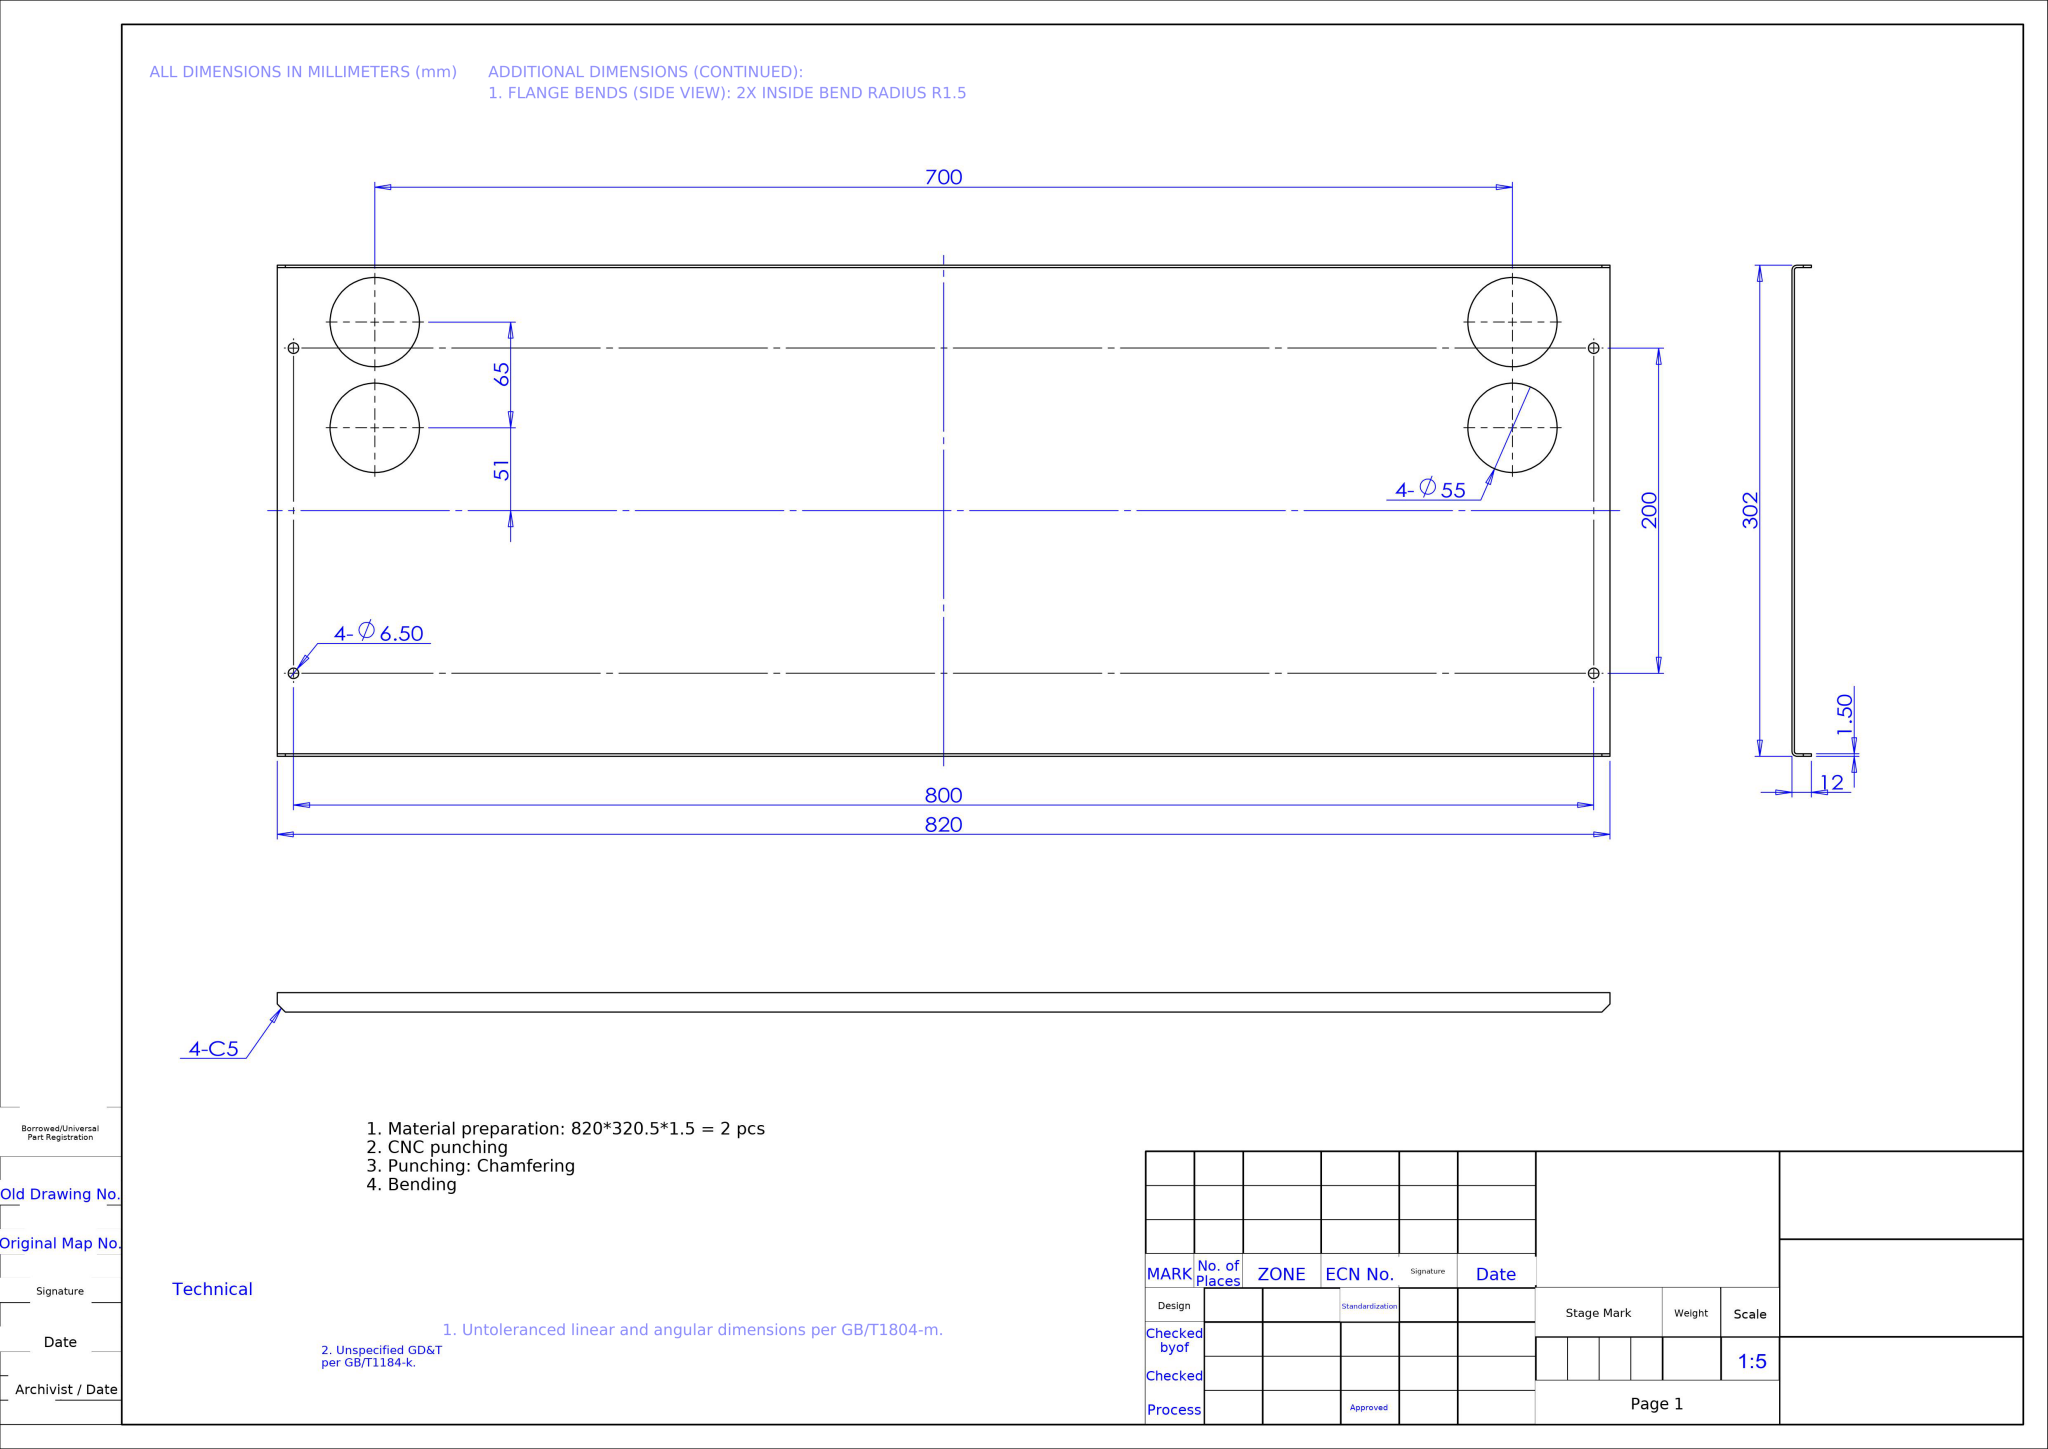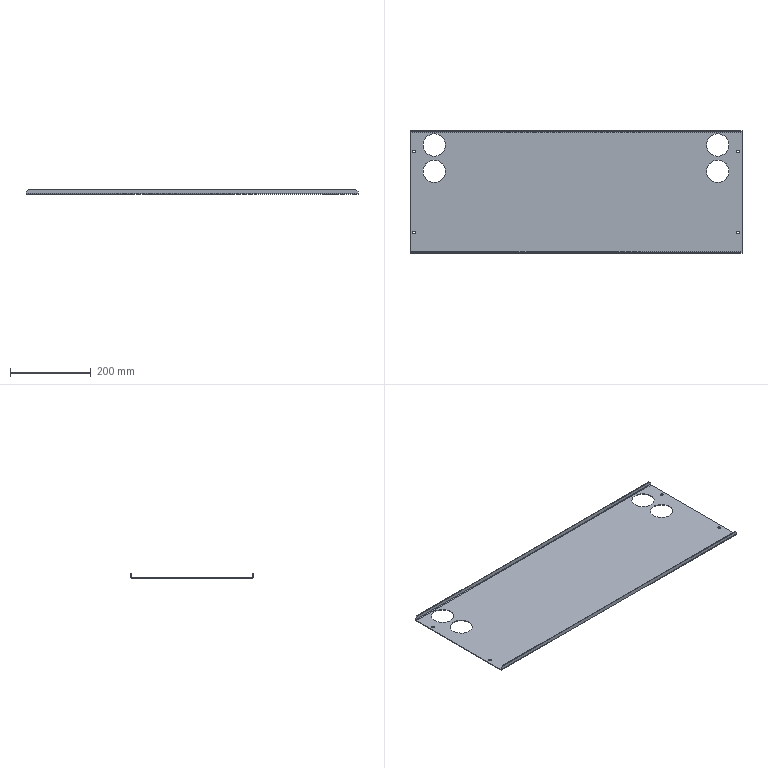Part | NX | mm | 1 solid | 42 faces | box 820 x 302 x 12 mm | volume 380385 mm3 | plane 22 | cylinder 20 | commonest cylinder face diameters 6.5 x8 55 x8 6 x2 3 x2